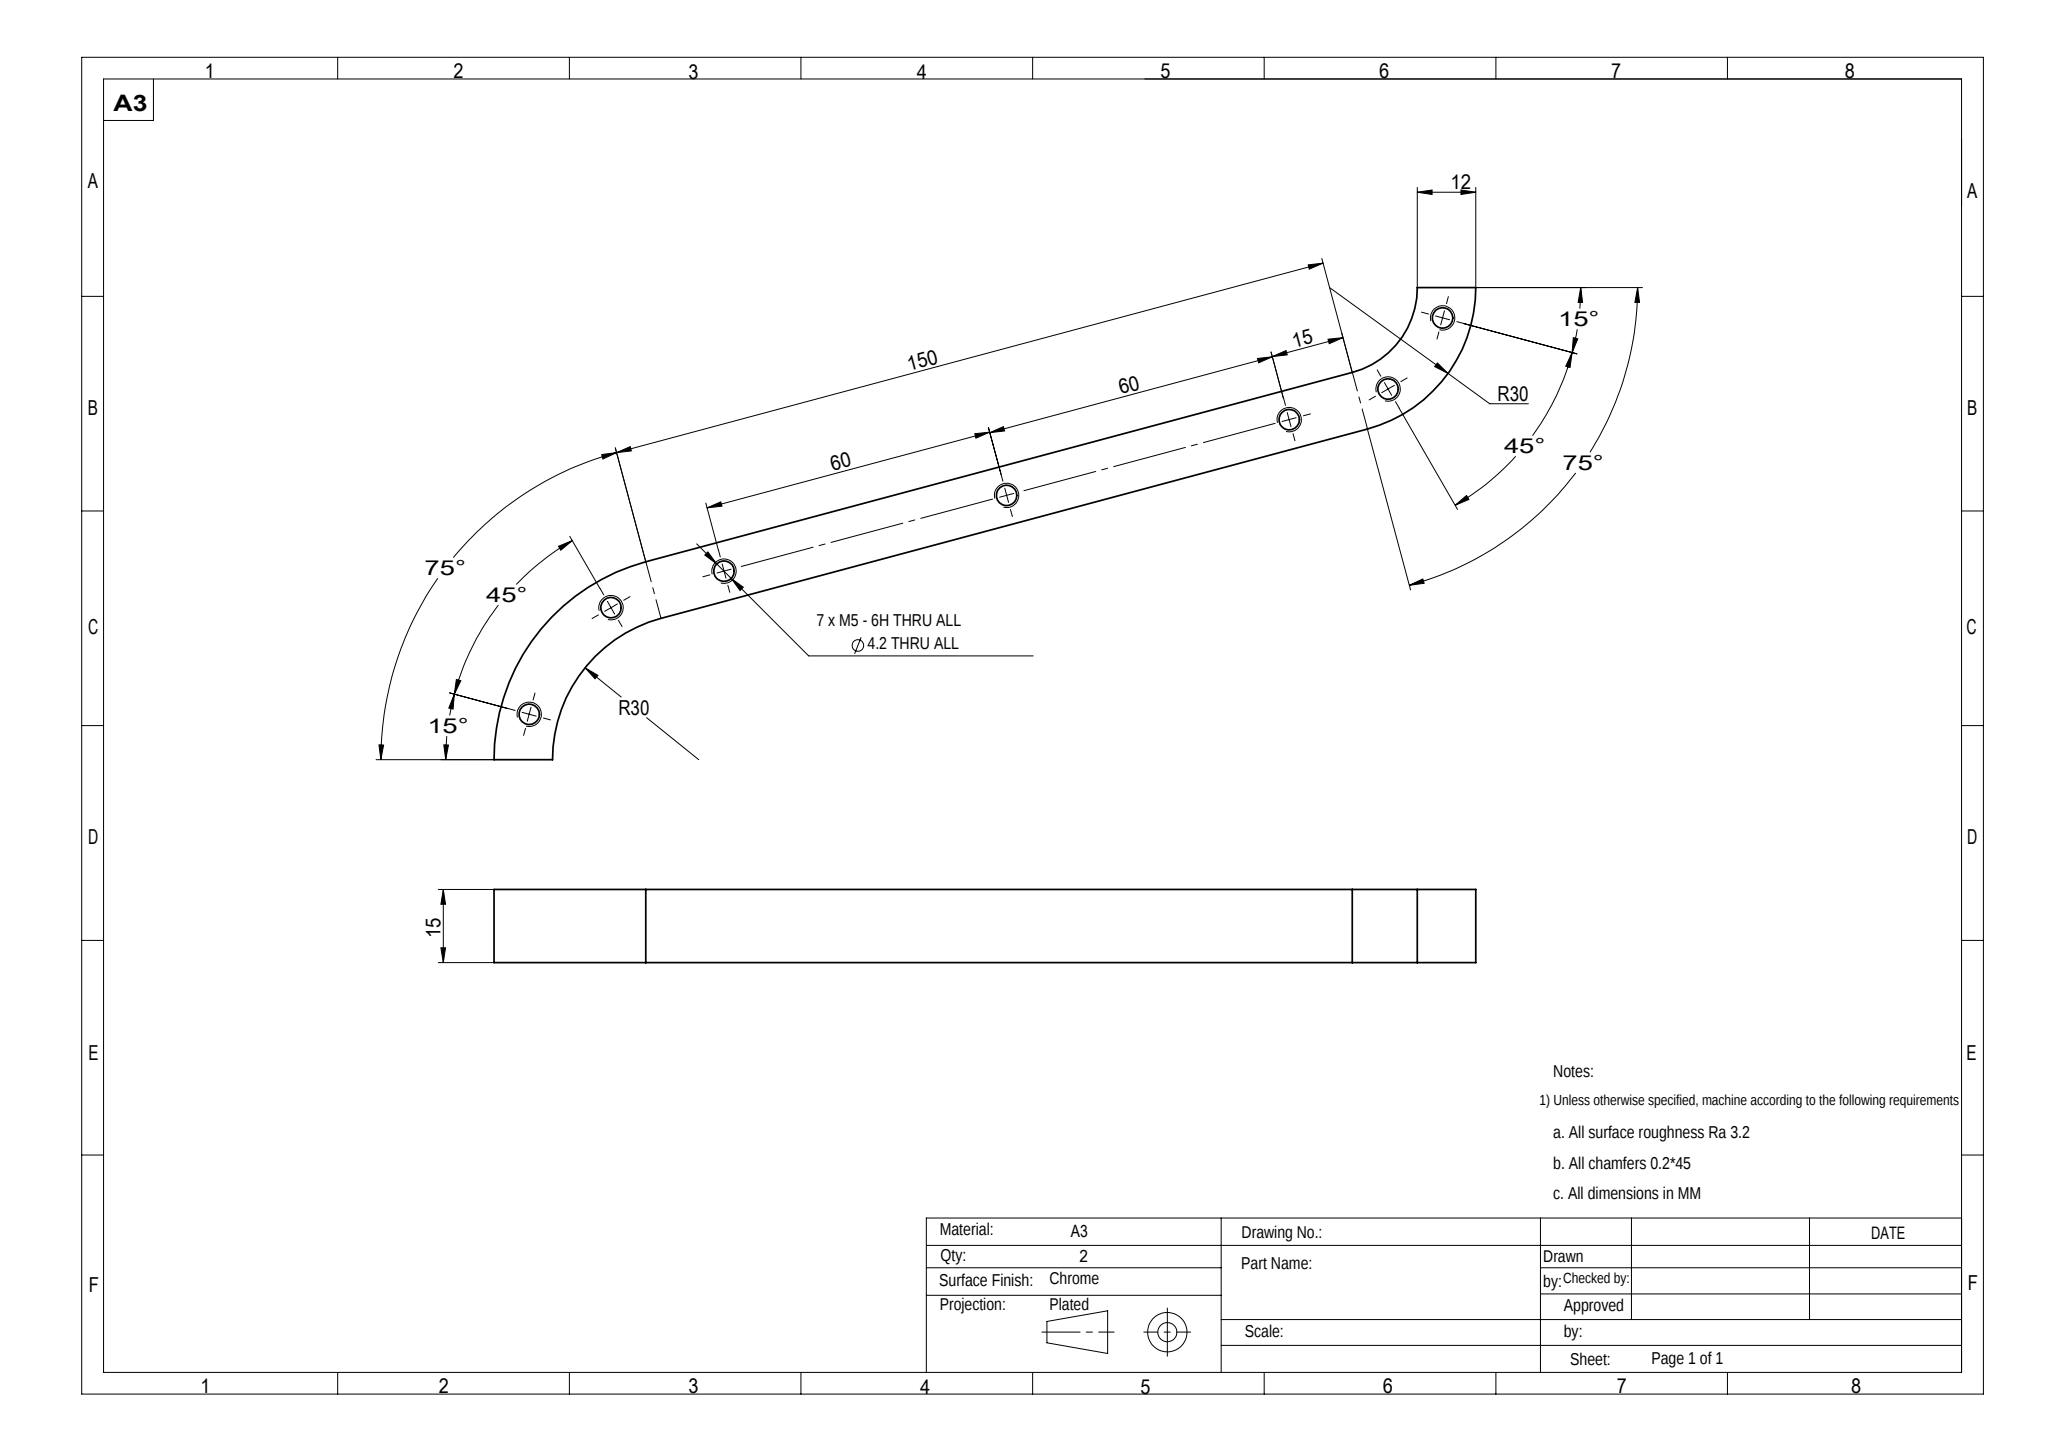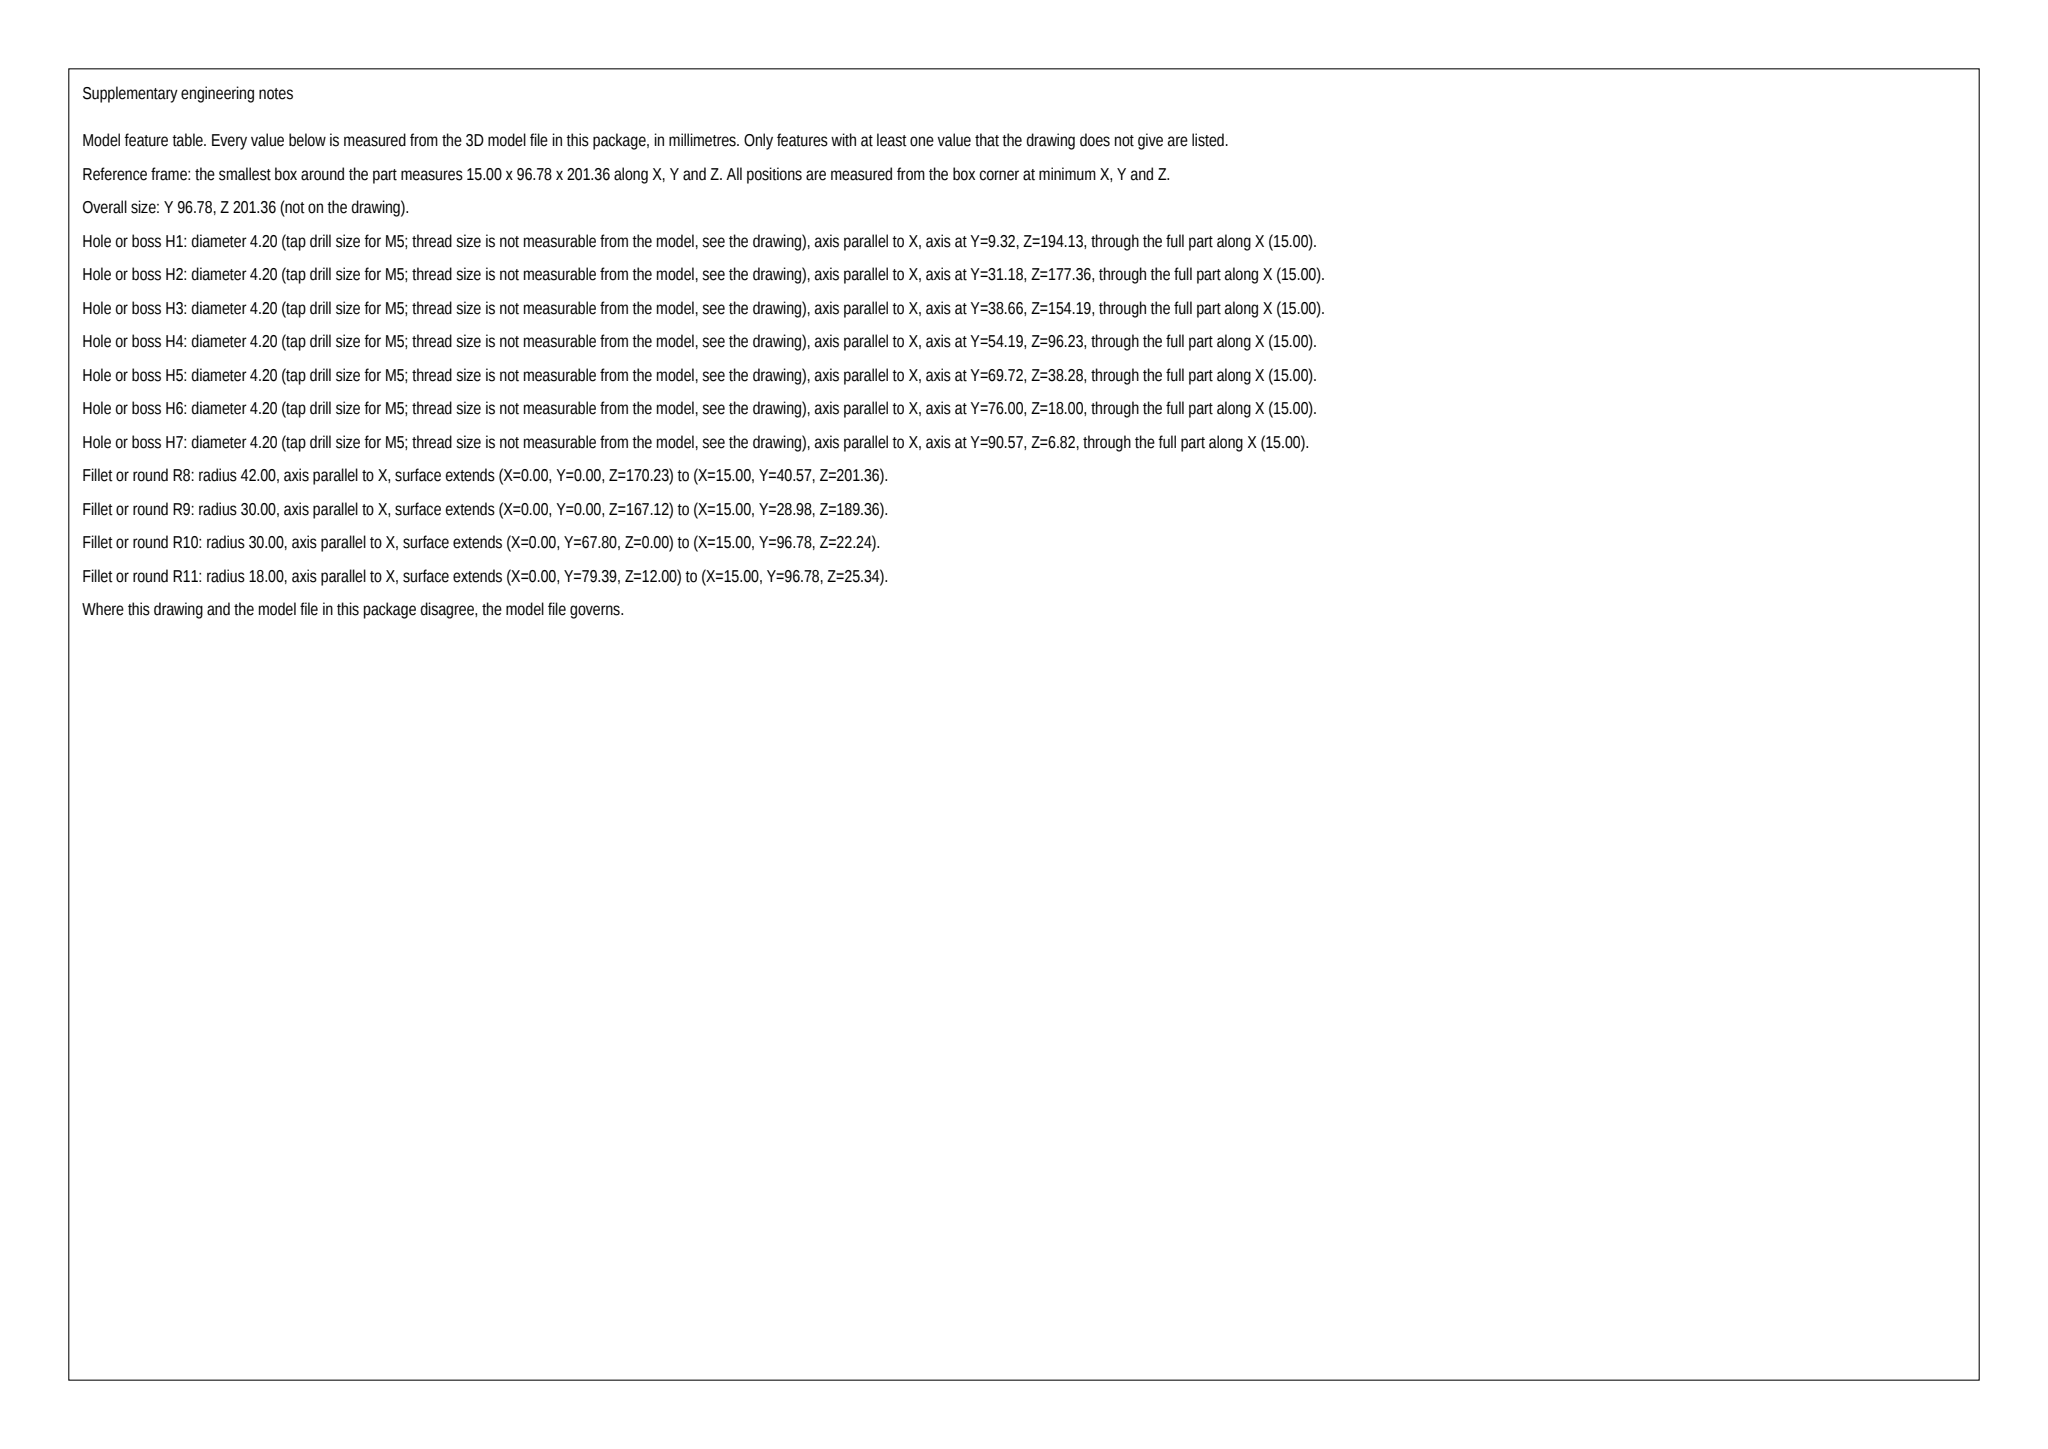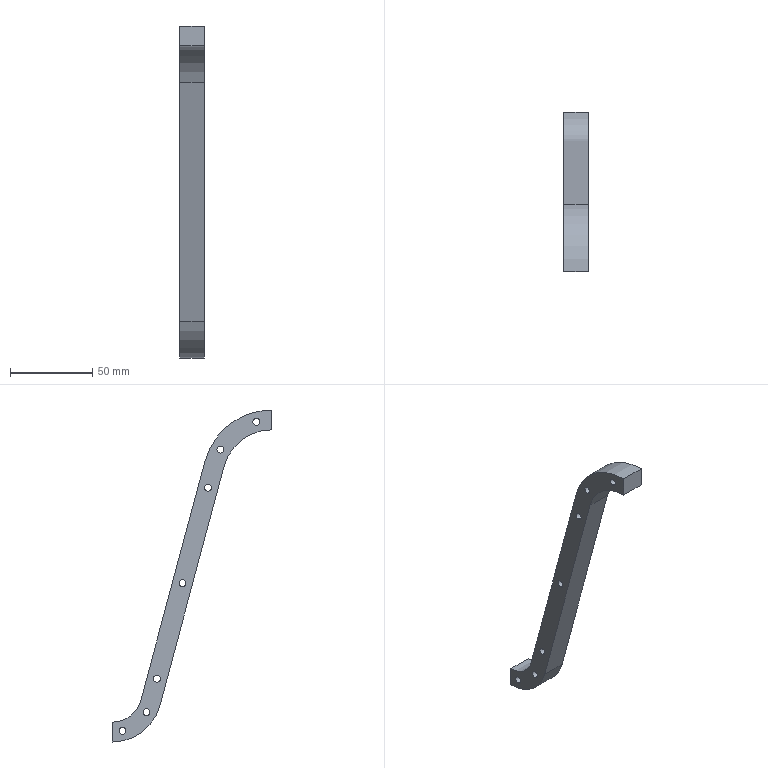Part | SolidWorks | mm | material A3 | 1 solid | 24 faces | box 15 x 96.78 x 201.36 mm | volume 39682 mm3 | cylinder 18 | plane 6 | commonest cylinder face diameters 4.2 x14 60 x2 36 x1 84 x1
Drawing notes:
LOWER BEND R18 INNER/R30 OUTER; UPPER BEND R30 INNER/R42 OUTER | from the solid: Concave dia 36 & convex dia 60 about (y96.8,z30); concave dia 60 & convex dia 84 about (y0,z159.4)
BEND HOLES AT 15 DEG & 60 DEG FROM END FACE ON 75 DEG ARC | from the solid: Holes (76.0,18.0) & (90.6,6.8) on R24 about (96.8,30); (9.3,194.1) & (31.2,177.4) on R36 about (0,159.4); 75 deg arcs
STRIP WIDTH 12 TYP THRU BENDS AND STRAIGHT SECTION | from the solid: Outer-inner radii diff: 30-18=12 and 42-30=12; end face extents z[189.4,201.4] and y[0,12]
7 X M5-6H THRU, MATL THK 15 | from the solid: 7 holes dia 4.2, x from 0.0 to 15.0 (plate thk 15)
TAP DRILL 7 X ::Ø4.2 THRU ALL | from the solid: 7 cylinders kind hole/bore dia 4.2 full thickness 0-15
build123d program:
from build123d import *

# Parameters (mm, degrees)
BOSS_EXTRUDE1_DEPTH = 7.5
M5_TAPPED_HOLE1_D   = 4.2


with BuildPart() as part:
    # Sketch1 → Boss-Extrude1 (new, symmetric)
    with BuildSketch(Plane(origin=(0, 0, 0), x_dir=(0, 0, -1), z_dir=(1, 0, 0))):
        with BuildLine():
            Line((-137.124, -67.801), (7.765, -28.978))
            ThreePointArc((7.765, -28.978), (23.801, -18.263), (30, 0))
            Line((30, 0), (18, 0))
            ThreePointArc((18, 0), (14.28, -10.958), (4.659, -17.387))
            Line((4.659, -17.387), (-140.23, -56.21))
            ThreePointArc((-140.23, -56.21), (-162.681, -71.21), (-171.36, -96.778))
            Line((-171.36, -96.778), (-159.36, -96.778))
            ThreePointArc((-159.36, -96.778), (-153.16, -78.516), (-137.124, -67.801))
        make_face()
    extrude(amount=BOSS_EXTRUDE1_DEPTH, both=True)

    # M5 Tapped Hole1 (through all)
    with Locations(Plane(origin=(7.5, 0, 0), x_dir=(0, 0, -1), z_dir=(1, 0, 0))):
        with Locations((23.182, -6.212), (12, -20.785), (-8.277, -27.065), (-66.233, -42.594), (-124.188, -58.123), (-147.36, -65.601), (-164.133, -87.461)):
            Hole(M5_TAPPED_HOLE1_D / 2)


solid = part.part
STEP:
#1=CARTESIAN_POINT('',(-7.5,-6.212,-21.082));
#2=VERTEX_POINT('',#1);
#3=CARTESIAN_POINT('',(-7.5,-6.212,-25.282));
#4=VERTEX_POINT('',#3);
#5=CARTESIAN_POINT('',(-7.5,-6.212,-23.182));
#6=DIRECTION('',(1.,0.,0.));
#7=DIRECTION('',(0.,0.,-1.));
#8=AXIS2_PLACEMENT_3D('',#5,#6,#7);
#9=CIRCLE('',#8,2.1);
#10=EDGE_CURVE('',#2,#4,#9,.T.);
#11=ORIENTED_EDGE('',*,*,#10,.F.);
#12=CARTESIAN_POINT('',(7.5,-6.212,-21.082));
#13=VERTEX_POINT('',#12);
#14=CARTESIAN_POINT('',(7.5,-6.212,-21.082));
#15=DIRECTION('',(1.,0.,0.));
#16=VECTOR('',#15,1000.);
#17=LINE('',#14,#16);
#18=EDGE_CURVE('',#2,#13,#17,.T.);
#19=ORIENTED_EDGE('',*,*,#18,.T.);
#20=CARTESIAN_POINT('',(7.5,-6.212,-25.282));
#21=VERTEX_POINT('',#20);
#22=CARTESIAN_POINT('',(7.5,-6.212,-23.182));
#23=DIRECTION('',(1.,0.,0.));
#24=DIRECTION('',(0.,0.,-1.));
#25=AXIS2_PLACEMENT_3D('',#22,#23,#24);
#26=CIRCLE('',#25,2.1);
#27=EDGE_CURVE('',#13,#21,#26,.T.);
#28=ORIENTED_EDGE('',*,*,#27,.T.);
#29=CARTESIAN_POINT('',(7.5,-6.212,-25.282));
#30=DIRECTION('',(1.,0.,0.));
#31=VECTOR('',#30,1000.);
#32=LINE('',#29,#31);
#33=EDGE_CURVE('',#4,#21,#32,.T.);
#34=ORIENTED_EDGE('',*,*,#33,.F.);
#35=EDGE_LOOP('',(#11,#19,#28,#34));
#36=FACE_OUTER_BOUND('',#35,.T.);
#37=CARTESIAN_POINT('',(7.5,-6.212,-23.182));
#38=DIRECTION('',(1.,0.,0.));
#39=DIRECTION('',(0.,0.,-1.));
#40=AXIS2_PLACEMENT_3D('',#37,#38,#39);
#41=CYLINDRICAL_SURFACE('',#40,2.1);
#42=ADVANCED_FACE('',(#36),#41,.F.);
#43=CARTESIAN_POINT('',(-7.5,-20.785,-9.9));
#44=VERTEX_POINT('',#43);
#45=CARTESIAN_POINT('',(-7.5,-20.785,-14.1));
#46=VERTEX_POINT('',#45);
#47=CARTESIAN_POINT('',(-7.5,-20.785,-12.));
#48=DIRECTION('',(1.,0.,0.));
#49=DIRECTION('',(0.,0.,-1.));
#50=AXIS2_PLACEMENT_3D('',#47,#48,#49);
#51=CIRCLE('',#50,2.1);
#52=EDGE_CURVE('',#44,#46,#51,.T.);
#53=ORIENTED_EDGE('',*,*,#52,.F.);
#54=CARTESIAN_POINT('',(7.5,-20.785,-9.9));
#55=VERTEX_POINT('',#54);
#56=CARTESIAN_POINT('',(7.5,-20.785,-9.9));
#57=DIRECTION('',(1.,0.,0.));
#58=VECTOR('',#57,1000.);
#59=LINE('',#56,#58);
#60=EDGE_CURVE('',#44,#55,#59,.T.);
#61=ORIENTED_EDGE('',*,*,#60,.T.);
#62=CARTESIAN_POINT('',(7.5,-20.785,-14.1));
#63=VERTEX_POINT('',#62);
#64=CARTESIAN_POINT('',(7.5,-20.785,-12.));
#65=DIRECTION('',(1.,0.,0.));
#66=DIRECTION('',(0.,0.,-1.));
#67=AXIS2_PLACEMENT_3D('',#64,#65,#66);
#68=CIRCLE('',#67,2.1);
#69=EDGE_CURVE('',#55,#63,#68,.T.);
#70=ORIENTED_EDGE('',*,*,#69,.T.);
#71=CARTESIAN_POINT('',(7.5,-20.785,-14.1));
#72=DIRECTION('',(1.,0.,0.));
#73=VECTOR('',#72,1000.);
#74=LINE('',#71,#73);
#75=EDGE_CURVE('',#46,#63,#74,.T.);
#76=ORIENTED_EDGE('',*,*,#75,.F.);
#77=EDGE_LOOP('',(#53,#61,#70,#76));
#78=FACE_OUTER_BOUND('',#77,.T.);
#79=CARTESIAN_POINT('',(7.5,-20.785,-12.));
#80=DIRECTION('',(1.,0.,0.));
#81=DIRECTION('',(0.,0.,-1.));
#82=AXIS2_PLACEMENT_3D('',#79,#80,#81);
#83=CYLINDRICAL_SURFACE('',#82,2.1);
#84=ADVANCED_FACE('',(#78),#83,.F.);
#85=CARTESIAN_POINT('',(-7.5,-27.065,10.377));
#86=VERTEX_POINT('',#85);
#87=CARTESIAN_POINT('',(-7.5,-27.065,6.177));
#88=VERTEX_POINT('',#87);
#89=CARTESIAN_POINT('',(-7.5,-27.065,8.277));
#90=DIRECTION('',(1.,0.,0.));
#91=DIRECTION('',(0.,0.,-1.));
#92=AXIS2_PLACEMENT_3D('',#89,#90,#91);
#93=CIRCLE('',#92,2.1);
#94=EDGE_CURVE('',#86,#88,#93,.T.);
#95=ORIENTED_EDGE('',*,*,#94,.F.);
#96=CARTESIAN_POINT('',(7.5,-27.065,10.377));
#97=VERTEX_POINT('',#96);
#98=CARTESIAN_POINT('',(7.5,-27.065,10.377));
#99=DIRECTION('',(1.,0.,0.));
#100=VECTOR('',#99,1000.);
#101=LINE('',#98,#100);
#102=EDGE_CURVE('',#86,#97,#101,.T.);
#103=ORIENTED_EDGE('',*,*,#102,.T.);
#104=CARTESIAN_POINT('',(7.5,-27.065,6.177));
#105=VERTEX_POINT('',#104);
#106=CARTESIAN_POINT('',(7.5,-27.065,8.277));
#107=DIRECTION('',(1.,0.,0.));
#108=DIRECTION('',(0.,0.,-1.));
#109=AXIS2_PLACEMENT_3D('',#106,#107,#108);
#110=CIRCLE('',#109,2.1);
#111=EDGE_CURVE('',#97,#105,#110,.T.);
#112=ORIENTED_EDGE('',*,*,#111,.T.);
#113=CARTESIAN_POINT('',(7.5,-27.065,6.177));
#114=DIRECTION('',(1.,0.,0.));
#115=VECTOR('',#114,1000.);
#116=LINE('',#113,#115);
#117=EDGE_CURVE('',#88,#105,#116,.T.);
#118=ORIENTED_EDGE('',*,*,#117,.F.);
#119=EDGE_LOOP('',(#95,#103,#112,#118));
#120=FACE_OUTER_BOUND('',#119,.T.);
#121=CARTESIAN_POINT('',(7.5,-27.065,8.277));
#122=DIRECTION('',(1.,0.,0.));
#123=DIRECTION('',(0.,0.,-1.));
#124=AXIS2_PLACEMENT_3D('',#121,#122,#123);
#125=CYLINDRICAL_SURFACE('',#124,2.1);
#126=ADVANCED_FACE('',(#120),#125,.F.);
#127=CARTESIAN_POINT('',(-7.5,-42.594,68.333));
#128=VERTEX_POINT('',#127);
#129=CARTESIAN_POINT('',(-7.5,-42.594,64.133));
#130=VERTEX_POINT('',#129);
#131=CARTESIAN_POINT('',(-7.5,-42.594,66.233));
#132=DIRECTION('',(1.,0.,0.));
#133=DIRECTION('',(0.,0.,-1.));
#134=AXIS2_PLACEMENT_3D('',#131,#132,#133);
#135=CIRCLE('',#134,2.1);
#136=EDGE_CURVE('',#128,#130,#135,.T.);
#137=ORIENTED_EDGE('',*,*,#136,.F.);
#138=CARTESIAN_POINT('',(7.5,-42.594,68.333));
#139=VERTEX_POINT('',#138);
#140=CARTESIAN_POINT('',(7.5,-42.594,68.333));
#141=DIRECTION('',(1.,0.,0.));
#142=VECTOR('',#141,1000.);
#143=LINE('',#140,#142);
#144=EDGE_CURVE('',#128,#139,#143,.T.);
#145=ORIENTED_EDGE('',*,*,#144,.T.);
#146=CARTESIAN_POINT('',(7.5,-42.594,64.133));
#147=VERTEX_POINT('',#146);
#148=CARTESIAN_POINT('',(7.5,-42.594,66.233));
#149=DIRECTION('',(1.,0.,0.));
#150=DIRECTION('',(0.,0.,-1.));
#151=AXIS2_PLACEMENT_3D('',#148,#149,#150);
#152=CIRCLE('',#151,2.1);
#153=EDGE_CURVE('',#139,#147,#152,.T.);
#154=ORIENTED_EDGE('',*,*,#153,.T.);
#155=CARTESIAN_POINT('',(7.5,-42.594,64.133));
#156=DIRECTION('',(1.,0.,0.));
#157=VECTOR('',#156,1000.);
#158=LINE('',#155,#157);
#159=EDGE_CURVE('',#130,#147,#158,.T.);
#160=ORIENTED_EDGE('',*,*,#159,.F.);
#161=EDGE_LOOP('',(#137,#145,#154,#160));
#162=FACE_OUTER_BOUND('',#161,.T.);
#163=CARTESIAN_POINT('',(7.5,-42.594,66.233));
#164=DIRECTION('',(1.,0.,0.));
#165=DIRECTION('',(0.,0.,-1.));
#166=AXIS2_PLACEMENT_3D('',#163,#164,#165);
#167=CYLINDRICAL_SURFACE('',#166,2.1);
#168=ADVANCED_FACE('',(#162),#167,.F.);
#169=CARTESIAN_POINT('',(-7.5,-58.123,126.288));
#170=VERTEX_POINT('',#169);
#171=CARTESIAN_POINT('',(-7.5,-58.123,122.088));
#172=VERTEX_POINT('',#171);
#173=CARTESIAN_POINT('',(-7.5,-58.123,124.188));
#174=DIRECTION('',(1.,0.,0.));
#175=DIRECTION('',(0.,0.,-1.));
#176=AXIS2_PLACEMENT_3D('',#173,#174,#175);
#177=CIRCLE('',#176,2.1);
#178=EDGE_CURVE('',#170,#172,#177,.T.);
#179=ORIENTED_EDGE('',*,*,#178,.F.);
#180=CARTESIAN_POINT('',(7.5,-58.123,126.288));
#181=VERTEX_POINT('',#180);
#182=CARTESIAN_POINT('',(7.5,-58.123,126.288));
#183=DIRECTION('',(1.,0.,0.));
#184=VECTOR('',#183,1000.);
#185=LINE('',#182,#184);
#186=EDGE_CURVE('',#170,#181,#185,.T.);
#187=ORIENTED_EDGE('',*,*,#186,.T.);
#188=CARTESIAN_POINT('',(7.5,-58.123,122.088));
#189=VERTEX_POINT('',#188);
#190=CARTESIAN_POINT('',(7.5,-58.123,124.188));
#191=DIRECTION('',(1.,0.,0.));
#192=DIRECTION('',(0.,0.,-1.));
#193=AXIS2_PLACEMENT_3D('',#190,#191,#192);
#194=CIRCLE('',#193,2.1);
#195=EDGE_CURVE('',#181,#189,#194,.T.);
#196=ORIENTED_EDGE('',*,*,#195,.T.);
#197=CARTESIAN_POINT('',(7.5,-58.123,122.088));
#198=DIRECTION('',(1.,0.,0.));
#199=VECTOR('',#198,1000.);
#200=LINE('',#197,#199);
#201=EDGE_CURVE('',#172,#189,#200,.T.);
#202=ORIENTED_EDGE('',*,*,#201,.F.);
#203=EDGE_LOOP('',(#179,#187,#196,#202));
#204=FACE_OUTER_BOUND('',#203,.T.);
#205=CARTESIAN_POINT('',(7.5,-58.123,124.188));
#206=DIRECTION('',(1.,0.,0.));
#207=DIRECTION('',(0.,0.,-1.));
#208=AXIS2_PLACEMENT_3D('',#205,#206,#207);
#209=CYLINDRICAL_SURFACE('',#208,2.1);
#210=ADVANCED_FACE('',(#204),#209,.F.);
#211=CARTESIAN_POINT('',(-7.5,-65.601,149.46));
#212=VERTEX_POINT('',#211);
#213=CARTESIAN_POINT('',(-7.5,-65.601,145.26));
#214=VERTEX_POINT('',#213);
#215=CARTESIAN_POINT('',(-7.5,-65.601,147.36));
#216=DIRECTION('',(1.,0.,0.));
#217=DIRECTION('',(0.,0.,-1.));
#218=AXIS2_PLACEMENT_3D('',#215,#216,#217);
#219=CIRCLE('',#218,2.1);
#220=EDGE_CURVE('',#212,#214,#219,.T.);
#221=ORIENTED_EDGE('',*,*,#220,.F.);
#222=CARTESIAN_POINT('',(7.5,-65.601,149.46));
#223=VERTEX_POINT('',#222);
#224=CARTESIAN_POINT('',(7.5,-65.601,149.46));
#225=DIRECTION('',(1.,0.,0.));
#226=VECTOR('',#225,1000.);
#227=LINE('',#224,#226);
#228=EDGE_CURVE('',#212,#223,#227,.T.);
#229=ORIENTED_EDGE('',*,*,#228,.T.);
#230=CARTESIAN_POINT('',(7.5,-65.601,145.26));
#231=VERTEX_POINT('',#230);
#232=CARTESIAN_POINT('',(7.5,-65.601,147.36));
#233=DIRECTION('',(1.,0.,0.));
#234=DIRECTION('',(0.,0.,-1.));
#235=AXIS2_PLACEMENT_3D('',#232,#233,#234);
#236=CIRCLE('',#235,2.1);
#237=EDGE_CURVE('',#223,#231,#236,.T.);
#238=ORIENTED_EDGE('',*,*,#237,.T.);
#239=CARTESIAN_POINT('',(7.5,-65.601,145.26));
#240=DIRECTION('',(1.,0.,0.));
#241=VECTOR('',#240,1000.);
#242=LINE('',#239,#241);
#243=EDGE_CURVE('',#214,#231,#242,.T.);
#244=ORIENTED_EDGE('',*,*,#243,.F.);
#245=EDGE_LOOP('',(#221,#229,#238,#244));
#246=FACE_OUTER_BOUND('',#245,.T.);
#247=CARTESIAN_POINT('',(7.5,-65.601,147.36));
#248=DIRECTION('',(1.,0.,0.));
#249=DIRECTION('',(0.,0.,-1.));
#250=AXIS2_PLACEMENT_3D('',#247,#248,#249);
#251=CYLINDRICAL_SURFACE('',#250,2.1);
#252=ADVANCED_FACE('',(#246),#251,.F.);
#253=CARTESIAN_POINT('',(-7.5,-87.461,166.233));
#254=VERTEX_POINT('',#253);
#255=CARTESIAN_POINT('',(-7.5,-87.461,162.033));
#256=VERTEX_POINT('',#255);
#257=CARTESIAN_POINT('',(-7.5,-87.461,164.133));
#258=DIRECTION('',(1.,0.,0.));
#259=DIRECTION('',(0.,0.,-1.));
#260=AXIS2_PLACEMENT_3D('',#257,#258,#259);
#261=CIRCLE('',#260,2.1);
#262=EDGE_CURVE('',#254,#256,#261,.T.);
#263=ORIENTED_EDGE('',*,*,#262,.F.);
#264=CARTESIAN_POINT('',(7.5,-87.461,166.233));
#265=VERTEX_POINT('',#264);
#266=CARTESIAN_POINT('',(7.5,-87.461,166.233));
#267=DIRECTION('',(1.,0.,0.));
#268=VECTOR('',#267,1000.);
#269=LINE('',#266,#268);
#270=EDGE_CURVE('',#254,#265,#269,.T.);
#271=ORIENTED_EDGE('',*,*,#270,.T.);
#272=CARTESIAN_POINT('',(7.5,-87.461,162.033));
#273=VERTEX_POINT('',#272);
#274=CARTESIAN_POINT('',(7.5,-87.461,164.133));
#275=DIRECTION('',(1.,0.,0.));
#276=DIRECTION('',(0.,0.,-1.));
#277=AXIS2_PLACEMENT_3D('',#274,#275,#276);
#278=CIRCLE('',#277,2.1);
#279=EDGE_CURVE('',#265,#273,#278,.T.);
#280=ORIENTED_EDGE('',*,*,#279,.T.);
#281=CARTESIAN_POINT('',(7.5,-87.461,162.033));
#282=DIRECTION('',(1.,0.,0.));
#283=VECTOR('',#282,1000.);
#284=LINE('',#281,#283);
#285=EDGE_CURVE('',#256,#273,#284,.T.);
#286=ORIENTED_EDGE('',*,*,#285,.F.);
#287=EDGE_LOOP('',(#263,#271,#280,#286));
#288=FACE_OUTER_BOUND('',#287,.T.);
#289=CARTESIAN_POINT('',(7.5,-87.461,164.133));
#290=DIRECTION('',(1.,0.,0.));
#291=DIRECTION('',(0.,0.,-1.));
#292=AXIS2_PLACEMENT_3D('',#289,#290,#291);
#293=CYLINDRICAL_SURFACE('',#292,2.1);
#294=ADVANCED_FACE('',(#288),#293,.F.);
#295=CARTESIAN_POINT('',(-7.5,-96.778,159.36));
#296=VERTEX_POINT('',#295);
#297=CARTESIAN_POINT('',(-7.5,-67.801,137.124));
#298=VERTEX_POINT('',#297);
#299=CARTESIAN_POINT('',(-7.5,-96.778,129.36));
#300=DIRECTION('',(-1.,0.,0.));
#301=DIRECTION('',(0.,0.,-1.));
#302=AXIS2_PLACEMENT_3D('',#299,#300,#301);
#303=CIRCLE('',#302,30.);
#304=EDGE_CURVE('',#296,#298,#303,.T.);
#305=ORIENTED_EDGE('',*,*,#304,.T.);
#306=CARTESIAN_POINT('',(7.5,-67.801,137.124));
#307=VERTEX_POINT('',#306);
#308=CARTESIAN_POINT('',(7.5,-67.801,137.124));
#309=DIRECTION('',(-1.,0.,0.));
#310=VECTOR('',#309,1000.);
#311=LINE('',#308,#310);
#312=EDGE_CURVE('',#307,#298,#311,.T.);
#313=ORIENTED_EDGE('',*,*,#312,.F.);
#314=CARTESIAN_POINT('',(7.5,-96.778,159.36));
#315=VERTEX_POINT('',#314);
#316=CARTESIAN_POINT('',(7.5,-96.778,129.36));
#317=DIRECTION('',(-1.,0.,0.));
#318=DIRECTION('',(0.,0.,-1.));
#319=AXIS2_PLACEMENT_3D('',#316,#317,#318);
#320=CIRCLE('',#319,30.);
#321=EDGE_CURVE('',#315,#307,#320,.T.);
#322=ORIENTED_EDGE('',*,*,#321,.F.);
#323=CARTESIAN_POINT('',(7.5,-96.778,159.36));
#324=DIRECTION('',(-1.,0.,0.));
#325=VECTOR('',#324,1000.);
#326=LINE('',#323,#325);
#327=EDGE_CURVE('',#315,#296,#326,.T.);
#328=ORIENTED_EDGE('',*,*,#327,.T.);
#329=EDGE_LOOP('',(#305,#313,#322,#328));
#330=FACE_OUTER_BOUND('',#329,.T.);
#331=CARTESIAN_POINT('',(7.5,-96.778,129.36));
#332=DIRECTION('',(-1.,0.,0.));
#333=DIRECTION('',(0.,0.,1.));
#334=AXIS2_PLACEMENT_3D('',#331,#332,#333);
#335=CYLINDRICAL_SURFACE('',#334,30.);
#336=ADVANCED_FACE('',(#330),#335,.F.);
#337=CARTESIAN_POINT('',(-7.5,-28.978,-7.765));
#338=VERTEX_POINT('',#337);
#339=CARTESIAN_POINT('',(-7.5,-67.801,137.124));
#340=DIRECTION('',(0.,0.2588,-0.9659));
#341=VECTOR('',#340,1000.);
#342=LINE('',#339,#341);
#343=EDGE_CURVE('',#298,#338,#342,.T.);
#344=ORIENTED_EDGE('',*,*,#343,.T.);
#345=CARTESIAN_POINT('',(7.5,-28.978,-7.765));
#346=VERTEX_POINT('',#345);
#347=CARTESIAN_POINT('',(7.5,-28.978,-7.765));
#348=DIRECTION('',(-1.,0.,0.));
#349=VECTOR('',#348,1000.);
#350=LINE('',#347,#349);
#351=EDGE_CURVE('',#346,#338,#350,.T.);
#352=ORIENTED_EDGE('',*,*,#351,.F.);
#353=CARTESIAN_POINT('',(7.5,-67.801,137.124));
#354=DIRECTION('',(0.,0.2588,-0.9659));
#355=VECTOR('',#354,1000.);
#356=LINE('',#353,#355);
#357=EDGE_CURVE('',#307,#346,#356,.T.);
#358=ORIENTED_EDGE('',*,*,#357,.F.);
#359=ORIENTED_EDGE('',*,*,#312,.T.);
#360=EDGE_LOOP('',(#344,#352,#358,#359));
#361=FACE_OUTER_BOUND('',#360,.T.);
#362=CARTESIAN_POINT('',(7.5,-67.801,137.124));
#363=DIRECTION('',(0.,0.9659,0.2588));
#364=DIRECTION('',(0.,-0.2588,0.9659));
#365=AXIS2_PLACEMENT_3D('',#362,#363,#364);
#366=PLANE('',#365);
#367=ADVANCED_FACE('',(#361),#366,.F.);
#368=CARTESIAN_POINT('',(-7.5,0.,-30.));
#369=VERTEX_POINT('',#368);
#370=CARTESIAN_POINT('',(-7.5,0.,0.));
#371=DIRECTION('',(1.,0.,0.));
#372=DIRECTION('',(0.,0.,-1.));
#373=AXIS2_PLACEMENT_3D('',#370,#371,#372);
#374=CIRCLE('',#373,30.);
#375=EDGE_CURVE('',#338,#369,#374,.T.);
#376=ORIENTED_EDGE('',*,*,#375,.T.);
#377=CARTESIAN_POINT('',(7.5,0.,-30.));
#378=VERTEX_POINT('',#377);
#379=CARTESIAN_POINT('',(7.5,0.,-30.));
#380=DIRECTION('',(-1.,0.,0.));
#381=VECTOR('',#380,1000.);
#382=LINE('',#379,#381);
#383=EDGE_CURVE('',#378,#369,#382,.T.);
#384=ORIENTED_EDGE('',*,*,#383,.F.);
#385=CARTESIAN_POINT('',(7.5,0.,0.));
#386=DIRECTION('',(1.,0.,0.));
#387=DIRECTION('',(0.,0.,-1.));
#388=AXIS2_PLACEMENT_3D('',#385,#386,#387);
#389=CIRCLE('',#388,30.);
#390=EDGE_CURVE('',#346,#378,#389,.T.);
#391=ORIENTED_EDGE('',*,*,#390,.F.);
#392=ORIENTED_EDGE('',*,*,#351,.T.);
#393=EDGE_LOOP('',(#376,#384,#391,#392));
#394=FACE_OUTER_BOUND('',#393,.T.);
#395=CARTESIAN_POINT('',(7.5,0.,0.));
#396=DIRECTION('',(-1.,0.,0.));
#397=DIRECTION('',(0.,0.,1.));
#398=AXIS2_PLACEMENT_3D('',#395,#396,#397);
#399=CYLINDRICAL_SURFACE('',#398,30.);
#400=ADVANCED_FACE('',(#394),#399,.T.);
#401=CARTESIAN_POINT('',(-7.5,-0.,-18.));
#402=VERTEX_POINT('',#401);
#403=CARTESIAN_POINT('',(-7.5,0.,-30.));
#404=DIRECTION('',(0.,-0.,1.));
#405=VECTOR('',#404,1000.);
#406=LINE('',#403,#405);
#407=EDGE_CURVE('',#369,#402,#406,.T.);
#408=ORIENTED_EDGE('',*,*,#407,.T.);
#409=CARTESIAN_POINT('',(7.5,-0.,-18.));
#410=VERTEX_POINT('',#409);
#411=CARTESIAN_POINT('',(7.5,-0.,-18.));
#412=DIRECTION('',(-1.,0.,0.));
#413=VECTOR('',#412,1000.);
#414=LINE('',#411,#413);
#415=EDGE_CURVE('',#410,#402,#414,.T.);
#416=ORIENTED_EDGE('',*,*,#415,.F.);
#417=CARTESIAN_POINT('',(7.5,0.,-30.));
#418=DIRECTION('',(0.,-0.,1.));
#419=VECTOR('',#418,1000.);
#420=LINE('',#417,#419);
#421=EDGE_CURVE('',#378,#410,#420,.T.);
#422=ORIENTED_EDGE('',*,*,#421,.F.);
#423=ORIENTED_EDGE('',*,*,#383,.T.);
#424=EDGE_LOOP('',(#408,#416,#422,#423));
#425=FACE_OUTER_BOUND('',#424,.T.);
#426=CARTESIAN_POINT('',(7.5,0.,-30.));
#427=DIRECTION('',(0.,-1.,-0.));
#428=DIRECTION('',(0.,0.,-1.));
#429=AXIS2_PLACEMENT_3D('',#426,#427,#428);
#430=PLANE('',#429);
#431=ADVANCED_FACE('',(#425),#430,.F.);
#432=CARTESIAN_POINT('',(-7.5,-17.387,-4.659));
#433=VERTEX_POINT('',#432);
#434=CARTESIAN_POINT('',(-7.5,0.,0.));
#435=DIRECTION('',(-1.,0.,0.));
#436=DIRECTION('',(0.,0.,1.));
#437=AXIS2_PLACEMENT_3D('',#434,#435,#436);
#438=CIRCLE('',#437,18.);
#439=EDGE_CURVE('',#402,#433,#438,.T.);
#440=ORIENTED_EDGE('',*,*,#439,.T.);
#441=CARTESIAN_POINT('',(7.5,-17.387,-4.659));
#442=VERTEX_POINT('',#441);
#443=CARTESIAN_POINT('',(7.5,-17.387,-4.659));
#444=DIRECTION('',(-1.,0.,0.));
#445=VECTOR('',#444,1000.);
#446=LINE('',#443,#445);
#447=EDGE_CURVE('',#442,#433,#446,.T.);
#448=ORIENTED_EDGE('',*,*,#447,.F.);
#449=CARTESIAN_POINT('',(7.5,0.,0.));
#450=DIRECTION('',(-1.,0.,0.));
#451=DIRECTION('',(0.,0.,1.));
#452=AXIS2_PLACEMENT_3D('',#449,#450,#451);
#453=CIRCLE('',#452,18.);
#454=EDGE_CURVE('',#410,#442,#453,.T.);
#455=ORIENTED_EDGE('',*,*,#454,.F.);
#456=ORIENTED_EDGE('',*,*,#415,.T.);
#457=EDGE_LOOP('',(#440,#448,#455,#456));
#458=FACE_OUTER_BOUND('',#457,.T.);
#459=CARTESIAN_POINT('',(7.5,0.,0.));
#460=DIRECTION('',(-1.,0.,0.));
#461=DIRECTION('',(0.,0.,1.));
#462=AXIS2_PLACEMENT_3D('',#459,#460,#461);
#463=CYLINDRICAL_SURFACE('',#462,18.);
#464=ADVANCED_FACE('',(#458),#463,.F.);
#465=CARTESIAN_POINT('',(-7.5,-56.21,140.23));
#466=VERTEX_POINT('',#465);
#467=CARTESIAN_POINT('',(-7.5,-17.387,-4.659));
#468=DIRECTION('',(0.,-0.2588,0.9659));
#469=VECTOR('',#468,1000.);
#470=LINE('',#467,#469);
#471=EDGE_CURVE('',#433,#466,#470,.T.);
#472=ORIENTED_EDGE('',*,*,#471,.T.);
#473=CARTESIAN_POINT('',(7.5,-56.21,140.23));
#474=VERTEX_POINT('',#473);
#475=CARTESIAN_POINT('',(7.5,-56.21,140.23));
#476=DIRECTION('',(-1.,0.,0.));
#477=VECTOR('',#476,1000.);
#478=LINE('',#475,#477);
#479=EDGE_CURVE('',#474,#466,#478,.T.);
#480=ORIENTED_EDGE('',*,*,#479,.F.);
#481=CARTESIAN_POINT('',(7.5,-17.387,-4.659));
#482=DIRECTION('',(0.,-0.2588,0.9659));
#483=VECTOR('',#482,1000.);
#484=LINE('',#481,#483);
#485=EDGE_CURVE('',#442,#474,#484,.T.);
#486=ORIENTED_EDGE('',*,*,#485,.F.);
#487=ORIENTED_EDGE('',*,*,#447,.T.);
#488=EDGE_LOOP('',(#472,#480,#486,#487));
#489=FACE_OUTER_BOUND('',#488,.T.);
#490=CARTESIAN_POINT('',(7.5,-17.387,-4.659));
#491=DIRECTION('',(0.,-0.9659,-0.2588));
#492=DIRECTION('',(0.,0.2588,-0.9659));
#493=AXIS2_PLACEMENT_3D('',#490,#491,#492);
#494=PLANE('',#493);
#495=ADVANCED_FACE('',(#489),#494,.F.);
#496=CARTESIAN_POINT('',(-7.5,-96.778,171.36));
#497=VERTEX_POINT('',#496);
#498=CARTESIAN_POINT('',(-7.5,-96.778,129.36));
#499=DIRECTION('',(1.,0.,0.));
#500=DIRECTION('',(0.,0.,-1.));
#501=AXIS2_PLACEMENT_3D('',#498,#499,#500);
#502=CIRCLE('',#501,42.);
#503=EDGE_CURVE('',#466,#497,#502,.T.);
#504=ORIENTED_EDGE('',*,*,#503,.T.);
#505=CARTESIAN_POINT('',(7.5,-96.778,171.36));
#506=VERTEX_POINT('',#505);
#507=CARTESIAN_POINT('',(7.5,-96.778,171.36));
#508=DIRECTION('',(-1.,0.,0.));
#509=VECTOR('',#508,1000.);
#510=LINE('',#507,#509);
#511=EDGE_CURVE('',#506,#497,#510,.T.);
#512=ORIENTED_EDGE('',*,*,#511,.F.);
#513=CARTESIAN_POINT('',(7.5,-96.778,129.36));
#514=DIRECTION('',(1.,0.,0.));
#515=DIRECTION('',(0.,0.,-1.));
#516=AXIS2_PLACEMENT_3D('',#513,#514,#515);
#517=CIRCLE('',#516,42.);
#518=EDGE_CURVE('',#474,#506,#517,.T.);
#519=ORIENTED_EDGE('',*,*,#518,.F.);
#520=ORIENTED_EDGE('',*,*,#479,.T.);
#521=EDGE_LOOP('',(#504,#512,#519,#520));
#522=FACE_OUTER_BOUND('',#521,.T.);
#523=CARTESIAN_POINT('',(7.5,-96.778,129.36));
#524=DIRECTION('',(-1.,0.,0.));
#525=DIRECTION('',(0.,0.,1.));
#526=AXIS2_PLACEMENT_3D('',#523,#524,#525);
#527=CYLINDRICAL_SURFACE('',#526,42.);
#528=ADVANCED_FACE('',(#522),#527,.T.);
#529=CARTESIAN_POINT('',(-7.5,-96.778,159.36));
#530=DIRECTION('',(0.,-0.,-1.));
#531=VECTOR('',#530,1000.);
#532=LINE('',#529,#531);
#533=EDGE_CURVE('',#497,#296,#532,.T.);
#534=ORIENTED_EDGE('',*,*,#533,.T.);
#535=ORIENTED_EDGE('',*,*,#327,.F.);
#536=CARTESIAN_POINT('',(7.5,-96.778,159.36));
#537=DIRECTION('',(0.,-0.,-1.));
#538=VECTOR('',#537,1000.);
#539=LINE('',#536,#538);
#540=EDGE_CURVE('',#506,#315,#539,.T.);
#541=ORIENTED_EDGE('',*,*,#540,.F.);
#542=ORIENTED_EDGE('',*,*,#511,.T.);
#543=EDGE_LOOP('',(#534,#535,#541,#542));
#544=FACE_OUTER_BOUND('',#543,.T.);
#545=CARTESIAN_POINT('',(7.5,-96.778,159.36));
#546=DIRECTION('',(0.,1.,-0.));
#547=DIRECTION('',(0.,0.,1.));
#548=AXIS2_PLACEMENT_3D('',#545,#546,#547);
#549=PLANE('',#548);
#550=ADVANCED_FACE('',(#544),#549,.F.);
#551=CARTESIAN_POINT('',(7.5,-6.212,-23.182));
#552=DIRECTION('',(1.,0.,0.));
#553=DIRECTION('',(0.,0.,-1.));
#554=AXIS2_PLACEMENT_3D('',#551,#552,#553);
#555=CIRCLE('',#554,2.1);
#556=EDGE_CURVE('',#21,#13,#555,.T.);
#557=ORIENTED_EDGE('',*,*,#556,.F.);
#558=ORIENTED_EDGE('',*,*,#27,.F.);
#559=EDGE_LOOP('',(#557,#558));
#560=FACE_BOUND('',#559,.T.);
#561=CARTESIAN_POINT('',(7.5,-20.785,-12.));
#562=DIRECTION('',(1.,0.,0.));
#563=DIRECTION('',(0.,0.,-1.));
#564=AXIS2_PLACEMENT_3D('',#561,#562,#563);
#565=CIRCLE('',#564,2.1);
#566=EDGE_CURVE('',#63,#55,#565,.T.);
#567=ORIENTED_EDGE('',*,*,#566,.F.);
#568=ORIENTED_EDGE('',*,*,#69,.F.);
#569=EDGE_LOOP('',(#567,#568));
#570=FACE_BOUND('',#569,.T.);
#571=CARTESIAN_POINT('',(7.5,-27.065,8.277));
#572=DIRECTION('',(1.,0.,0.));
#573=DIRECTION('',(0.,0.,-1.));
#574=AXIS2_PLACEMENT_3D('',#571,#572,#573);
#575=CIRCLE('',#574,2.1);
#576=EDGE_CURVE('',#105,#97,#575,.T.);
#577=ORIENTED_EDGE('',*,*,#576,.F.);
#578=ORIENTED_EDGE('',*,*,#111,.F.);
#579=EDGE_LOOP('',(#577,#578));
#580=FACE_BOUND('',#579,.T.);
#581=CARTESIAN_POINT('',(7.5,-42.594,66.233));
#582=DIRECTION('',(1.,0.,0.));
#583=DIRECTION('',(0.,0.,-1.));
#584=AXIS2_PLACEMENT_3D('',#581,#582,#583);
#585=CIRCLE('',#584,2.1);
#586=EDGE_CURVE('',#147,#139,#585,.T.);
#587=ORIENTED_EDGE('',*,*,#586,.F.);
#588=ORIENTED_EDGE('',*,*,#153,.F.);
#589=EDGE_LOOP('',(#587,#588));
#590=FACE_BOUND('',#589,.T.);
#591=CARTESIAN_POINT('',(7.5,-58.123,124.188));
#592=DIRECTION('',(1.,0.,0.));
#593=DIRECTION('',(0.,0.,-1.));
#594=AXIS2_PLACEMENT_3D('',#591,#592,#593);
#595=CIRCLE('',#594,2.1);
#596=EDGE_CURVE('',#189,#181,#595,.T.);
#597=ORIENTED_EDGE('',*,*,#596,.F.);
#598=ORIENTED_EDGE('',*,*,#195,.F.);
#599=EDGE_LOOP('',(#597,#598));
#600=FACE_BOUND('',#599,.T.);
#601=CARTESIAN_POINT('',(7.5,-65.601,147.36));
#602=DIRECTION('',(1.,0.,0.));
#603=DIRECTION('',(0.,0.,-1.));
#604=AXIS2_PLACEMENT_3D('',#601,#602,#603);
#605=CIRCLE('',#604,2.1);
#606=EDGE_CURVE('',#231,#223,#605,.T.);
#607=ORIENTED_EDGE('',*,*,#606,.F.);
#608=ORIENTED_EDGE('',*,*,#237,.F.);
#609=EDGE_LOOP('',(#607,#608));
#610=FACE_BOUND('',#609,.T.);
#611=CARTESIAN_POINT('',(7.5,-87.461,164.133));
#612=DIRECTION('',(1.,0.,0.));
#613=DIRECTION('',(0.,0.,-1.));
#614=AXIS2_PLACEMENT_3D('',#611,#612,#613);
#615=CIRCLE('',#614,2.1);
#616=EDGE_CURVE('',#273,#265,#615,.T.);
#617=ORIENTED_EDGE('',*,*,#616,.F.);
#618=ORIENTED_EDGE('',*,*,#279,.F.);
#619=EDGE_LOOP('',(#617,#618));
#620=FACE_BOUND('',#619,.T.);
#621=ORIENTED_EDGE('',*,*,#321,.T.);
#622=ORIENTED_EDGE('',*,*,#357,.T.);
#623=ORIENTED_EDGE('',*,*,#390,.T.);
#624=ORIENTED_EDGE('',*,*,#421,.T.);
#625=ORIENTED_EDGE('',*,*,#454,.T.);
#626=ORIENTED_EDGE('',*,*,#485,.T.);
#627=ORIENTED_EDGE('',*,*,#518,.T.);
#628=ORIENTED_EDGE('',*,*,#540,.T.);
#629=EDGE_LOOP('',(#621,#622,#623,#624,#625,#626,#627,#628));
#630=FACE_OUTER_BOUND('',#629,.T.);
#631=CARTESIAN_POINT('',(7.5,-96.778,129.36));
#632=DIRECTION('',(1.,0.,0.));
#633=DIRECTION('',(0.,0.,-1.));
#634=AXIS2_PLACEMENT_3D('',#631,#632,#633);
#635=PLANE('',#634);
#636=ADVANCED_FACE('',(#560,#570,#580,#590,#600,#610,#620,#630),#635,.T.);
#637=CARTESIAN_POINT('',(-7.5,-6.212,-23.182));
#638=DIRECTION('',(1.,0.,0.));
#639=DIRECTION('',(0.,0.,-1.));
#640=AXIS2_PLACEMENT_3D('',#637,#638,#639);
#641=CIRCLE('',#640,2.1);
#642=EDGE_CURVE('',#4,#2,#641,.T.);
#643=ORIENTED_EDGE('',*,*,#642,.T.);
#644=ORIENTED_EDGE('',*,*,#10,.T.);
#645=EDGE_LOOP('',(#643,#644));
#646=FACE_BOUND('',#645,.T.);
#647=CARTESIAN_POINT('',(-7.5,-20.785,-12.));
#648=DIRECTION('',(1.,0.,0.));
#649=DIRECTION('',(0.,0.,-1.));
#650=AXIS2_PLACEMENT_3D('',#647,#648,#649);
#651=CIRCLE('',#650,2.1);
#652=EDGE_CURVE('',#46,#44,#651,.T.);
#653=ORIENTED_EDGE('',*,*,#652,.T.);
#654=ORIENTED_EDGE('',*,*,#52,.T.);
#655=EDGE_LOOP('',(#653,#654));
#656=FACE_BOUND('',#655,.T.);
#657=CARTESIAN_POINT('',(-7.5,-27.065,8.277));
#658=DIRECTION('',(1.,0.,0.));
#659=DIRECTION('',(0.,0.,-1.));
#660=AXIS2_PLACEMENT_3D('',#657,#658,#659);
#661=CIRCLE('',#660,2.1);
#662=EDGE_CURVE('',#88,#86,#661,.T.);
#663=ORIENTED_EDGE('',*,*,#662,.T.);
#664=ORIENTED_EDGE('',*,*,#94,.T.);
#665=EDGE_LOOP('',(#663,#664));
#666=FACE_BOUND('',#665,.T.);
#667=CARTESIAN_POINT('',(-7.5,-42.594,66.233));
#668=DIRECTION('',(1.,0.,0.));
#669=DIRECTION('',(0.,0.,-1.));
#670=AXIS2_PLACEMENT_3D('',#667,#668,#669);
#671=CIRCLE('',#670,2.1);
#672=EDGE_CURVE('',#130,#128,#671,.T.);
#673=ORIENTED_EDGE('',*,*,#672,.T.);
#674=ORIENTED_EDGE('',*,*,#136,.T.);
#675=EDGE_LOOP('',(#673,#674));
#676=FACE_BOUND('',#675,.T.);
#677=CARTESIAN_POINT('',(-7.5,-58.123,124.188));
#678=DIRECTION('',(1.,0.,0.));
#679=DIRECTION('',(0.,0.,-1.));
#680=AXIS2_PLACEMENT_3D('',#677,#678,#679);
#681=CIRCLE('',#680,2.1);
#682=EDGE_CURVE('',#172,#170,#681,.T.);
#683=ORIENTED_EDGE('',*,*,#682,.T.);
#684=ORIENTED_EDGE('',*,*,#178,.T.);
#685=EDGE_LOOP('',(#683,#684));
#686=FACE_BOUND('',#685,.T.);
#687=CARTESIAN_POINT('',(-7.5,-65.601,147.36));
#688=DIRECTION('',(1.,0.,0.));
#689=DIRECTION('',(0.,0.,-1.));
#690=AXIS2_PLACEMENT_3D('',#687,#688,#689);
#691=CIRCLE('',#690,2.1);
#692=EDGE_CURVE('',#214,#212,#691,.T.);
#693=ORIENTED_EDGE('',*,*,#692,.T.);
#694=ORIENTED_EDGE('',*,*,#220,.T.);
#695=EDGE_LOOP('',(#693,#694));
#696=FACE_BOUND('',#695,.T.);
#697=CARTESIAN_POINT('',(-7.5,-87.461,164.133));
#698=DIRECTION('',(1.,0.,0.));
#699=DIRECTION('',(0.,0.,-1.));
#700=AXIS2_PLACEMENT_3D('',#697,#698,#699);
#701=CIRCLE('',#700,2.1);
#702=EDGE_CURVE('',#256,#254,#701,.T.);
#703=ORIENTED_EDGE('',*,*,#702,.T.);
#704=ORIENTED_EDGE('',*,*,#262,.T.);
#705=EDGE_LOOP('',(#703,#704));
#706=FACE_BOUND('',#705,.T.);
#707=ORIENTED_EDGE('',*,*,#304,.F.);
#708=ORIENTED_EDGE('',*,*,#533,.F.);
#709=ORIENTED_EDGE('',*,*,#503,.F.);
#710=ORIENTED_EDGE('',*,*,#471,.F.);
#711=ORIENTED_EDGE('',*,*,#439,.F.);
#712=ORIENTED_EDGE('',*,*,#407,.F.);
#713=ORIENTED_EDGE('',*,*,#375,.F.);
#714=ORIENTED_EDGE('',*,*,#343,.F.);
#715=EDGE_LOOP('',(#707,#708,#709,#710,#711,#712,#713,#714));
#716=FACE_OUTER_BOUND('',#715,.T.);
#717=CARTESIAN_POINT('',(-7.5,-96.778,129.36));
#718=DIRECTION('',(1.,0.,0.));
#719=DIRECTION('',(0.,0.,-1.));
#720=AXIS2_PLACEMENT_3D('',#717,#718,#719);
#721=PLANE('',#720);
#722=ADVANCED_FACE('',(#646,#656,#666,#676,#686,#696,#706,#716),#721,.F.);
#723=ORIENTED_EDGE('',*,*,#270,.F.);
#724=ORIENTED_EDGE('',*,*,#702,.F.);
#725=ORIENTED_EDGE('',*,*,#285,.T.);
#726=ORIENTED_EDGE('',*,*,#616,.T.);
#727=EDGE_LOOP('',(#723,#724,#725,#726));
#728=FACE_OUTER_BOUND('',#727,.T.);
#729=CARTESIAN_POINT('',(7.5,-87.461,164.133));
#730=DIRECTION('',(1.,0.,0.));
#731=DIRECTION('',(0.,0.,-1.));
#732=AXIS2_PLACEMENT_3D('',#729,#730,#731);
#733=CYLINDRICAL_SURFACE('',#732,2.1);
#734=ADVANCED_FACE('',(#728),#733,.F.);
#735=ORIENTED_EDGE('',*,*,#228,.F.);
#736=ORIENTED_EDGE('',*,*,#692,.F.);
#737=ORIENTED_EDGE('',*,*,#243,.T.);
#738=ORIENTED_EDGE('',*,*,#606,.T.);
#739=EDGE_LOOP('',(#735,#736,#737,#738));
#740=FACE_OUTER_BOUND('',#739,.T.);
#741=CARTESIAN_POINT('',(7.5,-65.601,147.36));
#742=DIRECTION('',(1.,0.,0.));
#743=DIRECTION('',(0.,0.,-1.));
#744=AXIS2_PLACEMENT_3D('',#741,#742,#743);
#745=CYLINDRICAL_SURFACE('',#744,2.1);
#746=ADVANCED_FACE('',(#740),#745,.F.);
#747=ORIENTED_EDGE('',*,*,#186,.F.);
#748=ORIENTED_EDGE('',*,*,#682,.F.);
#749=ORIENTED_EDGE('',*,*,#201,.T.);
#750=ORIENTED_EDGE('',*,*,#596,.T.);
#751=EDGE_LOOP('',(#747,#748,#749,#750));
#752=FACE_OUTER_BOUND('',#751,.T.);
#753=CARTESIAN_POINT('',(7.5,-58.123,124.188));
#754=DIRECTION('',(1.,0.,0.));
#755=DIRECTION('',(0.,0.,-1.));
#756=AXIS2_PLACEMENT_3D('',#753,#754,#755);
#757=CYLINDRICAL_SURFACE('',#756,2.1);
#758=ADVANCED_FACE('',(#752),#757,.F.);
#759=ORIENTED_EDGE('',*,*,#144,.F.);
#760=ORIENTED_EDGE('',*,*,#672,.F.);
#761=ORIENTED_EDGE('',*,*,#159,.T.);
#762=ORIENTED_EDGE('',*,*,#586,.T.);
#763=EDGE_LOOP('',(#759,#760,#761,#762));
#764=FACE_OUTER_BOUND('',#763,.T.);
#765=CARTESIAN_POINT('',(7.5,-42.594,66.233));
#766=DIRECTION('',(1.,0.,0.));
#767=DIRECTION('',(0.,0.,-1.));
#768=AXIS2_PLACEMENT_3D('',#765,#766,#767);
#769=CYLINDRICAL_SURFACE('',#768,2.1);
#770=ADVANCED_FACE('',(#764),#769,.F.);
#771=ORIENTED_EDGE('',*,*,#102,.F.);
#772=ORIENTED_EDGE('',*,*,#662,.F.);
#773=ORIENTED_EDGE('',*,*,#117,.T.);
#774=ORIENTED_EDGE('',*,*,#576,.T.);
#775=EDGE_LOOP('',(#771,#772,#773,#774));
#776=FACE_OUTER_BOUND('',#775,.T.);
#777=CARTESIAN_POINT('',(7.5,-27.065,8.277));
#778=DIRECTION('',(1.,0.,0.));
#779=DIRECTION('',(0.,0.,-1.));
#780=AXIS2_PLACEMENT_3D('',#777,#778,#779);
#781=CYLINDRICAL_SURFACE('',#780,2.1);
#782=ADVANCED_FACE('',(#776),#781,.F.);
#783=ORIENTED_EDGE('',*,*,#60,.F.);
#784=ORIENTED_EDGE('',*,*,#652,.F.);
#785=ORIENTED_EDGE('',*,*,#75,.T.);
#786=ORIENTED_EDGE('',*,*,#566,.T.);
#787=EDGE_LOOP('',(#783,#784,#785,#786));
#788=FACE_OUTER_BOUND('',#787,.T.);
#789=CARTESIAN_POINT('',(7.5,-20.785,-12.));
#790=DIRECTION('',(1.,0.,0.));
#791=DIRECTION('',(0.,0.,-1.));
#792=AXIS2_PLACEMENT_3D('',#789,#790,#791);
#793=CYLINDRICAL_SURFACE('',#792,2.1);
#794=ADVANCED_FACE('',(#788),#793,.F.);
#795=ORIENTED_EDGE('',*,*,#18,.F.);
#796=ORIENTED_EDGE('',*,*,#642,.F.);
#797=ORIENTED_EDGE('',*,*,#33,.T.);
#798=ORIENTED_EDGE('',*,*,#556,.T.);
#799=EDGE_LOOP('',(#795,#796,#797,#798));
#800=FACE_OUTER_BOUND('',#799,.T.);
#801=CARTESIAN_POINT('',(7.5,-6.212,-23.182));
#802=DIRECTION('',(1.,0.,0.));
#803=DIRECTION('',(0.,0.,-1.));
#804=AXIS2_PLACEMENT_3D('',#801,#802,#803);
#805=CYLINDRICAL_SURFACE('',#804,2.1);
#806=ADVANCED_FACE('',(#800),#805,.F.);
#807=CLOSED_SHELL('',(#42,#84,#126,#168,#210,#252,#294,#336,#367,#400,#431,#464,#495,#528,#550,#636,#722,#734,#746,#758,#770,#782,#794,#806));
#808=MANIFOLD_SOLID_BREP('',#807);
#809=CARTESIAN_POINT('',(0.,0.,0.));
#810=DIRECTION('',(0.,0.,1.));
#811=DIRECTION('',(1.,0.,0.));
#812=AXIS2_PLACEMENT_3D('',#809,#810,#811);
#813=(LENGTH_UNIT()NAMED_UNIT(*)SI_UNIT(.MILLI.,.METRE.));
#814=UNCERTAINTY_MEASURE_WITH_UNIT(LENGTH_MEASURE(0.00001),#813,'','');
#815=(NAMED_UNIT(*)PLANE_ANGLE_UNIT()SI_UNIT($,.RADIAN.));
#816=(NAMED_UNIT(*)SI_UNIT($,.STERADIAN.)SOLID_ANGLE_UNIT());
#817=(GEOMETRIC_REPRESENTATION_CONTEXT(3)GLOBAL_UNCERTAINTY_ASSIGNED_CONTEXT((#814))GLOBAL_UNIT_ASSIGNED_CONTEXT((#813,#815,#816))REPRESENTATION_CONTEXT('',''));
#818=ADVANCED_BREP_SHAPE_REPRESENTATION('',(#808,#812),#817);